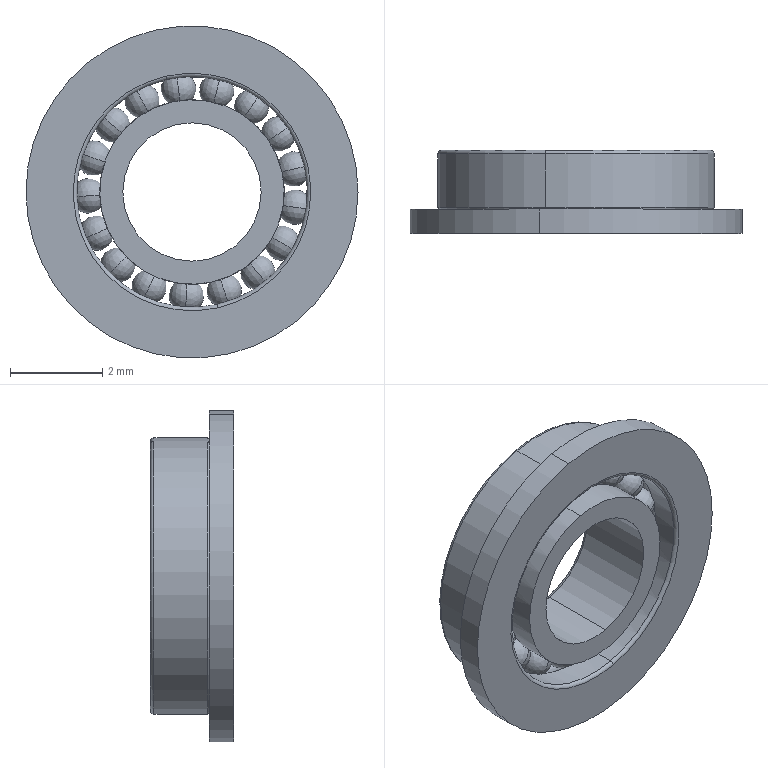Component | SolidWorks | miniature radial ball bearings gb1-1 | 1 solid | 117 faces | volume 34 mm3 | torus 64 | sphere 34 | cylinder 14 | plane 5 | commonest cylinder face diameters 5 x4 4 x4 7.2 x2 6 x2 3 x2